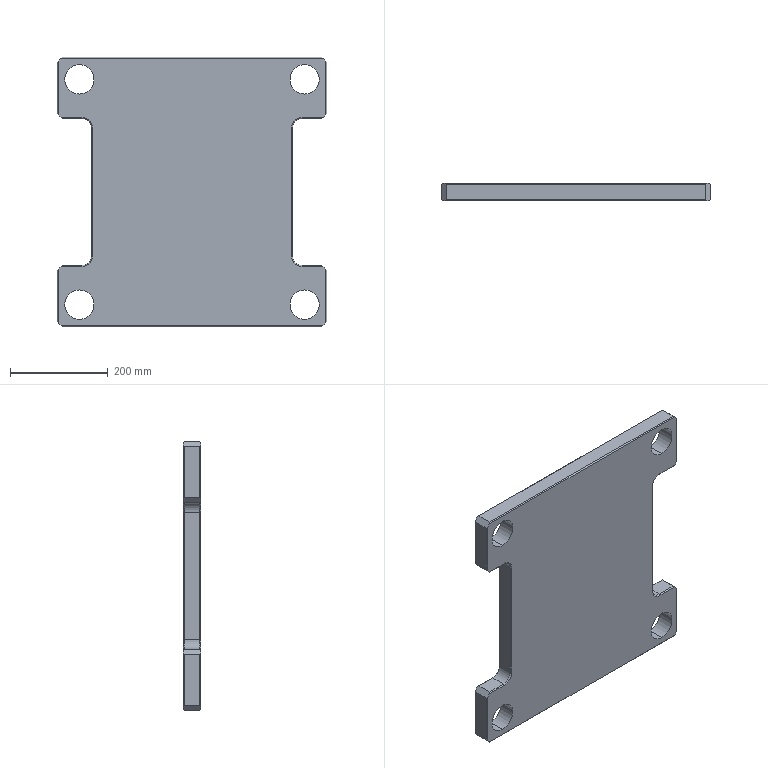Component | SolidWorks | UpperDieSlidingPlate-1 | 1 solid | 130 faces | volume 8698458 mm3 | plane 46 | cylinder 44 | cone 40 | commonest cylinder face diameters 6.8 x32 60 x8 40 x4